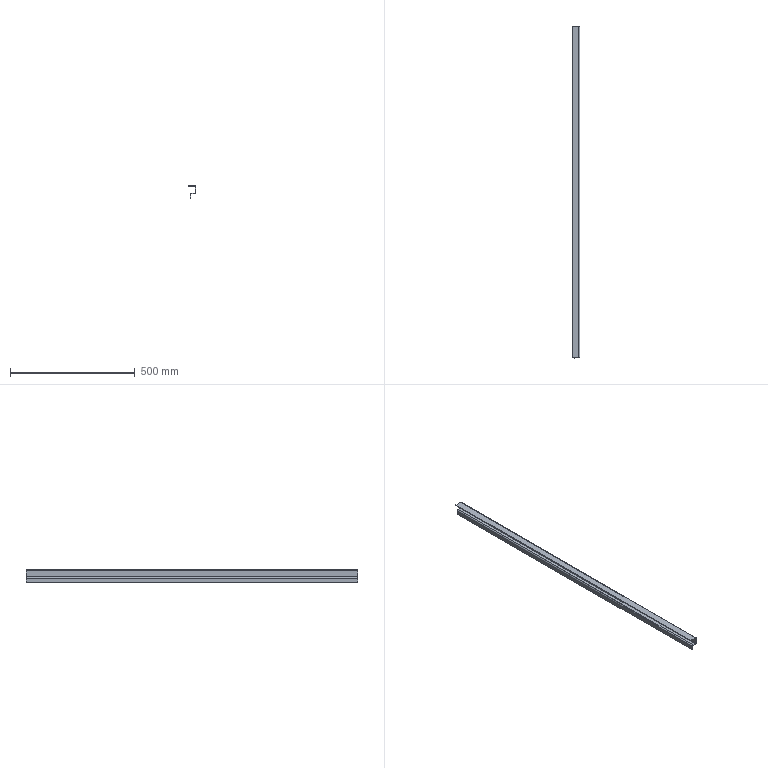Component | SolidWorks | BoxWelding-1_SupportPlate2.2-1 | 1 solid | 18 faces | box 31 x 1331 x 51 mm | volume 252490 mm3 | plane 12 | cylinder 6 | commonest cylinder face diameters 6 x3 10 x3
build123d program:
from build123d import *

# Parameters (mm, degrees)
EXTRUDE_THIN1_DEPTH = 665.5


with BuildPart() as part:
    # Sketch1 → Extrude-Thin1 (new, symmetric)
    with BuildSketch(Plane.XY):
        with BuildLine():
            Line((-1, 30), (-1, 4))
            ThreePointArc((-1, 4), (-1.879, 1.879), (-4, 1))
            Line((-4, 1), (-26, 1))
            ThreePointArc((-26, 1), (-28.121, 1.879), (-29, 4))
            Line((-29, 4), (-29, 16))
            ThreePointArc((-29, 16), (-30.464, 19.536), (-34, 21))
            Line((-34, 21), (-50, 21))
            Line((-50, 21), (-50, 19))
            Line((-50, 19), (-34, 19))
            ThreePointArc((-34, 19), (-31.879, 18.121), (-31, 16))
            Line((-31, 16), (-31, 4))
            ThreePointArc((-31, 4), (-29.536, 0.4645), (-26, -1))
            Line((-26, -1), (-4, -1))
            ThreePointArc((-4, -1), (-0.4645, 0.4645), (1, 4))
            Line((1, 4), (1, 30))
            Line((1, 30), (-1, 30))
        make_face()
    extrude(amount=EXTRUDE_THIN1_DEPTH, both=True)


solid = part.part

# Placed as in the assembly
solid = solid.moved(Location((450.622, 621.001, 379.013), (90, 0, 90)))
STEP:
#1=CARTESIAN_POINT('',(17.584,50.65,14.961));
#2=VERTEX_POINT('',#1);
#3=CARTESIAN_POINT('',(16.56,50.65,14.961));
#4=VERTEX_POINT('',#3);
#5=CARTESIAN_POINT('',(17.584,50.65,14.961));
#6=DIRECTION('',(-1.,-0.,-0.));
#7=VECTOR('',#6,39.37);
#8=LINE('',#5,#7);
#9=EDGE_CURVE('',#2,#4,#8,.T.);
#10=ORIENTED_EDGE('',*,*,#9,.T.);
#11=CARTESIAN_POINT('',(16.56,-1.752,14.961));
#12=VERTEX_POINT('',#11);
#13=CARTESIAN_POINT('',(16.56,-1.752,14.961));
#14=DIRECTION('',(-0.,1.,-0.));
#15=VECTOR('',#14,39.37);
#16=LINE('',#13,#15);
#17=EDGE_CURVE('',#12,#4,#16,.T.);
#18=ORIENTED_EDGE('',*,*,#17,.F.);
#19=CARTESIAN_POINT('',(17.584,-1.752,14.961));
#20=VERTEX_POINT('',#19);
#21=CARTESIAN_POINT('',(17.584,-1.752,14.961));
#22=DIRECTION('',(-1.,-0.,-0.));
#23=VECTOR('',#22,39.37);
#24=LINE('',#21,#23);
#25=EDGE_CURVE('',#20,#12,#24,.T.);
#26=ORIENTED_EDGE('',*,*,#25,.F.);
#27=CARTESIAN_POINT('',(17.584,-1.752,14.961));
#28=DIRECTION('',(-0.,1.,-0.));
#29=VECTOR('',#28,39.37);
#30=LINE('',#27,#29);
#31=EDGE_CURVE('',#20,#2,#30,.T.);
#32=ORIENTED_EDGE('',*,*,#31,.T.);
#33=EDGE_LOOP('',(#10,#18,#26,#32));
#34=FACE_OUTER_BOUND('',#33,.T.);
#35=CARTESIAN_POINT('',(17.584,-1.752,14.961));
#36=DIRECTION('',(0.,-0.,-1.));
#37=DIRECTION('',(0.,-1.,0.));
#38=AXIS2_PLACEMENT_3D('',#35,#36,#37);
#39=PLANE('',#38);
#40=ADVANCED_FACE('',(#34),#39,.F.);
#41=CARTESIAN_POINT('',(16.56,50.65,14.882));
#42=VERTEX_POINT('',#41);
#43=CARTESIAN_POINT('',(16.56,50.65,14.882));
#44=DIRECTION('',(-0.,0.,1.));
#45=VECTOR('',#44,39.37);
#46=LINE('',#43,#45);
#47=EDGE_CURVE('',#42,#4,#46,.T.);
#48=ORIENTED_EDGE('',*,*,#47,.F.);
#49=CARTESIAN_POINT('',(16.56,-1.752,14.882));
#50=VERTEX_POINT('',#49);
#51=CARTESIAN_POINT('',(16.56,-1.752,14.882));
#52=DIRECTION('',(-0.,1.,-0.));
#53=VECTOR('',#52,39.37);
#54=LINE('',#51,#53);
#55=EDGE_CURVE('',#50,#42,#54,.T.);
#56=ORIENTED_EDGE('',*,*,#55,.F.);
#57=CARTESIAN_POINT('',(16.56,-1.752,14.882));
#58=DIRECTION('',(-0.,0.,1.));
#59=VECTOR('',#58,39.37);
#60=LINE('',#57,#59);
#61=EDGE_CURVE('',#50,#12,#60,.T.);
#62=ORIENTED_EDGE('',*,*,#61,.T.);
#63=ORIENTED_EDGE('',*,*,#17,.T.);
#64=EDGE_LOOP('',(#48,#56,#62,#63));
#65=FACE_OUTER_BOUND('',#64,.T.);
#66=CARTESIAN_POINT('',(16.56,-1.752,14.882));
#67=DIRECTION('',(-1.,-0.,-0.));
#68=DIRECTION('',(0.,-1.,0.));
#69=AXIS2_PLACEMENT_3D('',#66,#67,#68);
#70=PLANE('',#69);
#71=ADVANCED_FACE('',(#65),#70,.T.);
#72=CARTESIAN_POINT('',(17.584,50.65,14.882));
#73=VERTEX_POINT('',#72);
#74=CARTESIAN_POINT('',(17.584,50.65,14.882));
#75=DIRECTION('',(-1.,-0.,-0.));
#76=VECTOR('',#75,39.37);
#77=LINE('',#74,#76);
#78=EDGE_CURVE('',#73,#42,#77,.T.);
#79=ORIENTED_EDGE('',*,*,#78,.F.);
#80=CARTESIAN_POINT('',(17.584,-1.752,14.882));
#81=VERTEX_POINT('',#80);
#82=CARTESIAN_POINT('',(17.584,-1.752,14.882));
#83=DIRECTION('',(-0.,1.,-0.));
#84=VECTOR('',#83,39.37);
#85=LINE('',#82,#84);
#86=EDGE_CURVE('',#81,#73,#85,.T.);
#87=ORIENTED_EDGE('',*,*,#86,.F.);
#88=CARTESIAN_POINT('',(17.584,-1.752,14.882));
#89=DIRECTION('',(-1.,-0.,-0.));
#90=VECTOR('',#89,39.37);
#91=LINE('',#88,#90);
#92=EDGE_CURVE('',#81,#50,#91,.T.);
#93=ORIENTED_EDGE('',*,*,#92,.T.);
#94=ORIENTED_EDGE('',*,*,#55,.T.);
#95=EDGE_LOOP('',(#79,#87,#93,#94));
#96=FACE_OUTER_BOUND('',#95,.T.);
#97=CARTESIAN_POINT('',(17.584,-1.752,14.882));
#98=DIRECTION('',(0.,-0.,-1.));
#99=DIRECTION('',(0.,-1.,0.));
#100=AXIS2_PLACEMENT_3D('',#97,#98,#99);
#101=PLANE('',#100);
#102=ADVANCED_FACE('',(#96),#101,.T.);
#103=CARTESIAN_POINT('',(17.702,50.65,14.764));
#104=VERTEX_POINT('',#103);
#105=CARTESIAN_POINT('',(17.584,50.65,14.764));
#106=DIRECTION('',(0.,-1.,0.));
#107=DIRECTION('',(0.,0.,1.));
#108=AXIS2_PLACEMENT_3D('',#105,#106,#107);
#109=CIRCLE('',#108,0.1181);
#110=EDGE_CURVE('',#104,#73,#109,.T.);
#111=ORIENTED_EDGE('',*,*,#110,.F.);
#112=CARTESIAN_POINT('',(17.702,-1.752,14.764));
#113=VERTEX_POINT('',#112);
#114=CARTESIAN_POINT('',(17.702,-1.752,14.764));
#115=DIRECTION('',(-0.,1.,-0.));
#116=VECTOR('',#115,39.37);
#117=LINE('',#114,#116);
#118=EDGE_CURVE('',#113,#104,#117,.T.);
#119=ORIENTED_EDGE('',*,*,#118,.F.);
#120=CARTESIAN_POINT('',(17.584,-1.752,14.764));
#121=DIRECTION('',(0.,-1.,0.));
#122=DIRECTION('',(0.,0.,1.));
#123=AXIS2_PLACEMENT_3D('',#120,#121,#122);
#124=CIRCLE('',#123,0.1181);
#125=EDGE_CURVE('',#113,#81,#124,.T.);
#126=ORIENTED_EDGE('',*,*,#125,.T.);
#127=ORIENTED_EDGE('',*,*,#86,.T.);
#128=EDGE_LOOP('',(#111,#119,#126,#127));
#129=FACE_OUTER_BOUND('',#128,.T.);
#130=CARTESIAN_POINT('',(17.584,-1.752,14.764));
#131=DIRECTION('',(-0.,1.,-0.));
#132=DIRECTION('',(0.,-0.,-1.));
#133=AXIS2_PLACEMENT_3D('',#130,#131,#132);
#134=CYLINDRICAL_SURFACE('',#133,0.1181);
#135=ADVANCED_FACE('',(#129),#134,.F.);
#136=CARTESIAN_POINT('',(17.702,50.65,13.898));
#137=VERTEX_POINT('',#136);
#138=CARTESIAN_POINT('',(17.702,50.65,14.764));
#139=DIRECTION('',(-0.,0.,1.));
#140=VECTOR('',#139,39.37);
#141=LINE('',#138,#140);
#142=EDGE_CURVE('',#137,#104,#141,.T.);
#143=ORIENTED_EDGE('',*,*,#142,.F.);
#144=CARTESIAN_POINT('',(17.702,-1.752,13.898));
#145=VERTEX_POINT('',#144);
#146=CARTESIAN_POINT('',(17.702,-1.752,13.898));
#147=DIRECTION('',(-0.,1.,-0.));
#148=VECTOR('',#147,39.37);
#149=LINE('',#146,#148);
#150=EDGE_CURVE('',#145,#137,#149,.T.);
#151=ORIENTED_EDGE('',*,*,#150,.F.);
#152=CARTESIAN_POINT('',(17.702,-1.752,14.764));
#153=DIRECTION('',(-0.,0.,1.));
#154=VECTOR('',#153,39.37);
#155=LINE('',#152,#154);
#156=EDGE_CURVE('',#145,#113,#155,.T.);
#157=ORIENTED_EDGE('',*,*,#156,.T.);
#158=ORIENTED_EDGE('',*,*,#118,.T.);
#159=EDGE_LOOP('',(#143,#151,#157,#158));
#160=FACE_OUTER_BOUND('',#159,.T.);
#161=CARTESIAN_POINT('',(17.702,-1.752,14.764));
#162=DIRECTION('',(-1.,-0.,-0.));
#163=DIRECTION('',(0.,-1.,0.));
#164=AXIS2_PLACEMENT_3D('',#161,#162,#163);
#165=PLANE('',#164);
#166=ADVANCED_FACE('',(#160),#165,.T.);
#167=CARTESIAN_POINT('',(17.584,50.65,13.78));
#168=VERTEX_POINT('',#167);
#169=CARTESIAN_POINT('',(17.584,50.65,13.898));
#170=DIRECTION('',(0.,-1.,0.));
#171=DIRECTION('',(0.,0.,1.));
#172=AXIS2_PLACEMENT_3D('',#169,#170,#171);
#173=CIRCLE('',#172,0.1181);
#174=EDGE_CURVE('',#168,#137,#173,.T.);
#175=ORIENTED_EDGE('',*,*,#174,.F.);
#176=CARTESIAN_POINT('',(17.584,-1.752,13.78));
#177=VERTEX_POINT('',#176);
#178=CARTESIAN_POINT('',(17.584,-1.752,13.78));
#179=DIRECTION('',(-0.,1.,-0.));
#180=VECTOR('',#179,39.37);
#181=LINE('',#178,#180);
#182=EDGE_CURVE('',#177,#168,#181,.T.);
#183=ORIENTED_EDGE('',*,*,#182,.F.);
#184=CARTESIAN_POINT('',(17.584,-1.752,13.898));
#185=DIRECTION('',(0.,-1.,0.));
#186=DIRECTION('',(0.,0.,1.));
#187=AXIS2_PLACEMENT_3D('',#184,#185,#186);
#188=CIRCLE('',#187,0.1181);
#189=EDGE_CURVE('',#177,#145,#188,.T.);
#190=ORIENTED_EDGE('',*,*,#189,.T.);
#191=ORIENTED_EDGE('',*,*,#150,.T.);
#192=EDGE_LOOP('',(#175,#183,#190,#191));
#193=FACE_OUTER_BOUND('',#192,.T.);
#194=CARTESIAN_POINT('',(17.584,-1.752,13.898));
#195=DIRECTION('',(-0.,1.,-0.));
#196=DIRECTION('',(0.,-0.,-1.));
#197=AXIS2_PLACEMENT_3D('',#194,#195,#196);
#198=CYLINDRICAL_SURFACE('',#197,0.1181);
#199=ADVANCED_FACE('',(#193),#198,.F.);
#200=CARTESIAN_POINT('',(17.111,50.65,13.78));
#201=VERTEX_POINT('',#200);
#202=CARTESIAN_POINT('',(17.584,50.65,13.78));
#203=DIRECTION('',(1.,0.,0.));
#204=VECTOR('',#203,39.37);
#205=LINE('',#202,#204);
#206=EDGE_CURVE('',#201,#168,#205,.T.);
#207=ORIENTED_EDGE('',*,*,#206,.F.);
#208=CARTESIAN_POINT('',(17.111,-1.752,13.78));
#209=VERTEX_POINT('',#208);
#210=CARTESIAN_POINT('',(17.111,-1.752,13.78));
#211=DIRECTION('',(-0.,1.,-0.));
#212=VECTOR('',#211,39.37);
#213=LINE('',#210,#212);
#214=EDGE_CURVE('',#209,#201,#213,.T.);
#215=ORIENTED_EDGE('',*,*,#214,.F.);
#216=CARTESIAN_POINT('',(17.584,-1.752,13.78));
#217=DIRECTION('',(1.,0.,0.));
#218=VECTOR('',#217,39.37);
#219=LINE('',#216,#218);
#220=EDGE_CURVE('',#209,#177,#219,.T.);
#221=ORIENTED_EDGE('',*,*,#220,.T.);
#222=ORIENTED_EDGE('',*,*,#182,.T.);
#223=EDGE_LOOP('',(#207,#215,#221,#222));
#224=FACE_OUTER_BOUND('',#223,.T.);
#225=CARTESIAN_POINT('',(17.584,-1.752,13.78));
#226=DIRECTION('',(-0.,0.,1.));
#227=DIRECTION('',(-0.,1.,-0.));
#228=AXIS2_PLACEMENT_3D('',#225,#226,#227);
#229=PLANE('',#228);
#230=ADVANCED_FACE('',(#224),#229,.T.);
#231=CARTESIAN_POINT('',(16.914,50.65,13.583));
#232=VERTEX_POINT('',#231);
#233=CARTESIAN_POINT('',(17.111,50.65,13.583));
#234=DIRECTION('',(-0.,1.,-0.));
#235=DIRECTION('',(0.,0.,1.));
#236=AXIS2_PLACEMENT_3D('',#233,#234,#235);
#237=CIRCLE('',#236,0.1969);
#238=EDGE_CURVE('',#232,#201,#237,.T.);
#239=ORIENTED_EDGE('',*,*,#238,.F.);
#240=CARTESIAN_POINT('',(16.914,-1.752,13.583));
#241=VERTEX_POINT('',#240);
#242=CARTESIAN_POINT('',(16.914,-1.752,13.583));
#243=DIRECTION('',(-0.,1.,-0.));
#244=VECTOR('',#243,39.37);
#245=LINE('',#242,#244);
#246=EDGE_CURVE('',#241,#232,#245,.T.);
#247=ORIENTED_EDGE('',*,*,#246,.F.);
#248=CARTESIAN_POINT('',(17.111,-1.752,13.583));
#249=DIRECTION('',(-0.,1.,-0.));
#250=DIRECTION('',(-0.,0.,1.));
#251=AXIS2_PLACEMENT_3D('',#248,#249,#250);
#252=CIRCLE('',#251,0.1969);
#253=EDGE_CURVE('',#241,#209,#252,.T.);
#254=ORIENTED_EDGE('',*,*,#253,.T.);
#255=ORIENTED_EDGE('',*,*,#214,.T.);
#256=EDGE_LOOP('',(#239,#247,#254,#255));
#257=FACE_OUTER_BOUND('',#256,.T.);
#258=CARTESIAN_POINT('',(17.111,-1.752,13.583));
#259=DIRECTION('',(-0.,1.,-0.));
#260=DIRECTION('',(0.,-0.,-1.));
#261=AXIS2_PLACEMENT_3D('',#258,#259,#260);
#262=CYLINDRICAL_SURFACE('',#261,0.1969);
#263=ADVANCED_FACE('',(#257),#262,.T.);
#264=CARTESIAN_POINT('',(16.914,50.65,12.953));
#265=VERTEX_POINT('',#264);
#266=CARTESIAN_POINT('',(16.914,50.65,13.583));
#267=DIRECTION('',(-0.,0.,1.));
#268=VECTOR('',#267,39.37);
#269=LINE('',#266,#268);
#270=EDGE_CURVE('',#265,#232,#269,.T.);
#271=ORIENTED_EDGE('',*,*,#270,.F.);
#272=CARTESIAN_POINT('',(16.914,-1.752,12.953));
#273=VERTEX_POINT('',#272);
#274=CARTESIAN_POINT('',(16.914,-1.752,12.953));
#275=DIRECTION('',(-0.,1.,-0.));
#276=VECTOR('',#275,39.37);
#277=LINE('',#274,#276);
#278=EDGE_CURVE('',#273,#265,#277,.T.);
#279=ORIENTED_EDGE('',*,*,#278,.F.);
#280=CARTESIAN_POINT('',(16.914,-1.752,13.583));
#281=DIRECTION('',(-0.,0.,1.));
#282=VECTOR('',#281,39.37);
#283=LINE('',#280,#282);
#284=EDGE_CURVE('',#273,#241,#283,.T.);
#285=ORIENTED_EDGE('',*,*,#284,.T.);
#286=ORIENTED_EDGE('',*,*,#246,.T.);
#287=EDGE_LOOP('',(#271,#279,#285,#286));
#288=FACE_OUTER_BOUND('',#287,.T.);
#289=CARTESIAN_POINT('',(16.914,-1.752,13.583));
#290=DIRECTION('',(-1.,-0.,-0.));
#291=DIRECTION('',(0.,-0.,-1.));
#292=AXIS2_PLACEMENT_3D('',#289,#290,#291);
#293=PLANE('',#292);
#294=ADVANCED_FACE('',(#288),#293,.T.);
#295=CARTESIAN_POINT('',(16.993,50.65,12.953));
#296=VERTEX_POINT('',#295);
#297=CARTESIAN_POINT('',(16.993,50.65,12.953));
#298=DIRECTION('',(-1.,-0.,-0.));
#299=VECTOR('',#298,39.37);
#300=LINE('',#297,#299);
#301=EDGE_CURVE('',#296,#265,#300,.T.);
#302=ORIENTED_EDGE('',*,*,#301,.F.);
#303=CARTESIAN_POINT('',(16.993,-1.752,12.953));
#304=VERTEX_POINT('',#303);
#305=CARTESIAN_POINT('',(16.993,-1.752,12.953));
#306=DIRECTION('',(-0.,1.,-0.));
#307=VECTOR('',#306,39.37);
#308=LINE('',#305,#307);
#309=EDGE_CURVE('',#304,#296,#308,.T.);
#310=ORIENTED_EDGE('',*,*,#309,.F.);
#311=CARTESIAN_POINT('',(16.993,-1.752,12.953));
#312=DIRECTION('',(-1.,-0.,-0.));
#313=VECTOR('',#312,39.37);
#314=LINE('',#311,#313);
#315=EDGE_CURVE('',#304,#273,#314,.T.);
#316=ORIENTED_EDGE('',*,*,#315,.T.);
#317=ORIENTED_EDGE('',*,*,#278,.T.);
#318=EDGE_LOOP('',(#302,#310,#316,#317));
#319=FACE_OUTER_BOUND('',#318,.T.);
#320=CARTESIAN_POINT('',(16.993,-1.752,12.953));
#321=DIRECTION('',(0.,-0.,-1.));
#322=DIRECTION('',(0.,-1.,0.));
#323=AXIS2_PLACEMENT_3D('',#320,#321,#322);
#324=PLANE('',#323);
#325=ADVANCED_FACE('',(#319),#324,.T.);
#326=CARTESIAN_POINT('',(16.993,50.65,13.583));
#327=VERTEX_POINT('',#326);
#328=CARTESIAN_POINT('',(16.993,50.65,13.583));
#329=DIRECTION('',(-0.,0.,1.));
#330=VECTOR('',#329,39.37);
#331=LINE('',#328,#330);
#332=EDGE_CURVE('',#296,#327,#331,.T.);
#333=ORIENTED_EDGE('',*,*,#332,.T.);
#334=CARTESIAN_POINT('',(16.993,-1.752,13.583));
#335=VERTEX_POINT('',#334);
#336=CARTESIAN_POINT('',(16.993,-1.752,13.583));
#337=DIRECTION('',(-0.,1.,-0.));
#338=VECTOR('',#337,39.37);
#339=LINE('',#336,#338);
#340=EDGE_CURVE('',#335,#327,#339,.T.);
#341=ORIENTED_EDGE('',*,*,#340,.F.);
#342=CARTESIAN_POINT('',(16.993,-1.752,13.583));
#343=DIRECTION('',(-0.,0.,1.));
#344=VECTOR('',#343,39.37);
#345=LINE('',#342,#344);
#346=EDGE_CURVE('',#304,#335,#345,.T.);
#347=ORIENTED_EDGE('',*,*,#346,.F.);
#348=ORIENTED_EDGE('',*,*,#309,.T.);
#349=EDGE_LOOP('',(#333,#341,#347,#348));
#350=FACE_OUTER_BOUND('',#349,.T.);
#351=CARTESIAN_POINT('',(16.993,-1.752,13.583));
#352=DIRECTION('',(-1.,-0.,-0.));
#353=DIRECTION('',(0.,-0.,-1.));
#354=AXIS2_PLACEMENT_3D('',#351,#352,#353);
#355=PLANE('',#354);
#356=ADVANCED_FACE('',(#350),#355,.F.);
#357=CARTESIAN_POINT('',(17.111,50.65,13.701));
#358=VERTEX_POINT('',#357);
#359=CARTESIAN_POINT('',(17.111,50.65,13.583));
#360=DIRECTION('',(-0.,1.,-0.));
#361=DIRECTION('',(0.,0.,1.));
#362=AXIS2_PLACEMENT_3D('',#359,#360,#361);
#363=CIRCLE('',#362,0.1181);
#364=EDGE_CURVE('',#327,#358,#363,.T.);
#365=ORIENTED_EDGE('',*,*,#364,.T.);
#366=CARTESIAN_POINT('',(17.111,-1.752,13.701));
#367=VERTEX_POINT('',#366);
#368=CARTESIAN_POINT('',(17.111,-1.752,13.701));
#369=DIRECTION('',(-0.,1.,-0.));
#370=VECTOR('',#369,39.37);
#371=LINE('',#368,#370);
#372=EDGE_CURVE('',#367,#358,#371,.T.);
#373=ORIENTED_EDGE('',*,*,#372,.F.);
#374=CARTESIAN_POINT('',(17.111,-1.752,13.583));
#375=DIRECTION('',(-0.,1.,-0.));
#376=DIRECTION('',(-0.,0.,1.));
#377=AXIS2_PLACEMENT_3D('',#374,#375,#376);
#378=CIRCLE('',#377,0.1181);
#379=EDGE_CURVE('',#335,#367,#378,.T.);
#380=ORIENTED_EDGE('',*,*,#379,.F.);
#381=ORIENTED_EDGE('',*,*,#340,.T.);
#382=EDGE_LOOP('',(#365,#373,#380,#381));
#383=FACE_OUTER_BOUND('',#382,.T.);
#384=CARTESIAN_POINT('',(17.111,-1.752,13.583));
#385=DIRECTION('',(-0.,1.,-0.));
#386=DIRECTION('',(0.,-0.,-1.));
#387=AXIS2_PLACEMENT_3D('',#384,#385,#386);
#388=CYLINDRICAL_SURFACE('',#387,0.1181);
#389=ADVANCED_FACE('',(#383),#388,.F.);
#390=CARTESIAN_POINT('',(17.584,50.65,13.701));
#391=VERTEX_POINT('',#390);
#392=CARTESIAN_POINT('',(17.584,50.65,13.701));
#393=DIRECTION('',(1.,0.,0.));
#394=VECTOR('',#393,39.37);
#395=LINE('',#392,#394);
#396=EDGE_CURVE('',#358,#391,#395,.T.);
#397=ORIENTED_EDGE('',*,*,#396,.T.);
#398=CARTESIAN_POINT('',(17.584,-1.752,13.701));
#399=VERTEX_POINT('',#398);
#400=CARTESIAN_POINT('',(17.584,-1.752,13.701));
#401=DIRECTION('',(-0.,1.,-0.));
#402=VECTOR('',#401,39.37);
#403=LINE('',#400,#402);
#404=EDGE_CURVE('',#399,#391,#403,.T.);
#405=ORIENTED_EDGE('',*,*,#404,.F.);
#406=CARTESIAN_POINT('',(17.584,-1.752,13.701));
#407=DIRECTION('',(1.,0.,0.));
#408=VECTOR('',#407,39.37);
#409=LINE('',#406,#408);
#410=EDGE_CURVE('',#367,#399,#409,.T.);
#411=ORIENTED_EDGE('',*,*,#410,.F.);
#412=ORIENTED_EDGE('',*,*,#372,.T.);
#413=EDGE_LOOP('',(#397,#405,#411,#412));
#414=FACE_OUTER_BOUND('',#413,.T.);
#415=CARTESIAN_POINT('',(17.584,-1.752,13.701));
#416=DIRECTION('',(-0.,0.,1.));
#417=DIRECTION('',(-0.,1.,-0.));
#418=AXIS2_PLACEMENT_3D('',#415,#416,#417);
#419=PLANE('',#418);
#420=ADVANCED_FACE('',(#414),#419,.F.);
#421=CARTESIAN_POINT('',(17.78,50.65,13.898));
#422=VERTEX_POINT('',#421);
#423=CARTESIAN_POINT('',(17.584,50.65,13.898));
#424=DIRECTION('',(0.,-1.,0.));
#425=DIRECTION('',(0.,0.,1.));
#426=AXIS2_PLACEMENT_3D('',#423,#424,#425);
#427=CIRCLE('',#426,0.1969);
#428=EDGE_CURVE('',#391,#422,#427,.T.);
#429=ORIENTED_EDGE('',*,*,#428,.T.);
#430=CARTESIAN_POINT('',(17.78,-1.752,13.898));
#431=VERTEX_POINT('',#430);
#432=CARTESIAN_POINT('',(17.78,-1.752,13.898));
#433=DIRECTION('',(-0.,1.,-0.));
#434=VECTOR('',#433,39.37);
#435=LINE('',#432,#434);
#436=EDGE_CURVE('',#431,#422,#435,.T.);
#437=ORIENTED_EDGE('',*,*,#436,.F.);
#438=CARTESIAN_POINT('',(17.584,-1.752,13.898));
#439=DIRECTION('',(0.,-1.,0.));
#440=DIRECTION('',(0.,0.,1.));
#441=AXIS2_PLACEMENT_3D('',#438,#439,#440);
#442=CIRCLE('',#441,0.1969);
#443=EDGE_CURVE('',#399,#431,#442,.T.);
#444=ORIENTED_EDGE('',*,*,#443,.F.);
#445=ORIENTED_EDGE('',*,*,#404,.T.);
#446=EDGE_LOOP('',(#429,#437,#444,#445));
#447=FACE_OUTER_BOUND('',#446,.T.);
#448=CARTESIAN_POINT('',(17.584,-1.752,13.898));
#449=DIRECTION('',(-0.,1.,-0.));
#450=DIRECTION('',(0.,-0.,-1.));
#451=AXIS2_PLACEMENT_3D('',#448,#449,#450);
#452=CYLINDRICAL_SURFACE('',#451,0.1969);
#453=ADVANCED_FACE('',(#447),#452,.T.);
#454=CARTESIAN_POINT('',(17.78,50.65,14.764));
#455=VERTEX_POINT('',#454);
#456=CARTESIAN_POINT('',(17.78,50.65,14.764));
#457=DIRECTION('',(-0.,0.,1.));
#458=VECTOR('',#457,39.37);
#459=LINE('',#456,#458);
#460=EDGE_CURVE('',#422,#455,#459,.T.);
#461=ORIENTED_EDGE('',*,*,#460,.T.);
#462=CARTESIAN_POINT('',(17.78,-1.752,14.764));
#463=VERTEX_POINT('',#462);
#464=CARTESIAN_POINT('',(17.78,-1.752,14.764));
#465=DIRECTION('',(-0.,1.,-0.));
#466=VECTOR('',#465,39.37);
#467=LINE('',#464,#466);
#468=EDGE_CURVE('',#463,#455,#467,.T.);
#469=ORIENTED_EDGE('',*,*,#468,.F.);
#470=CARTESIAN_POINT('',(17.78,-1.752,14.764));
#471=DIRECTION('',(-0.,0.,1.));
#472=VECTOR('',#471,39.37);
#473=LINE('',#470,#472);
#474=EDGE_CURVE('',#431,#463,#473,.T.);
#475=ORIENTED_EDGE('',*,*,#474,.F.);
#476=ORIENTED_EDGE('',*,*,#436,.T.);
#477=EDGE_LOOP('',(#461,#469,#475,#476));
#478=FACE_OUTER_BOUND('',#477,.T.);
#479=CARTESIAN_POINT('',(17.78,-1.752,14.764));
#480=DIRECTION('',(-1.,-0.,-0.));
#481=DIRECTION('',(0.,-1.,0.));
#482=AXIS2_PLACEMENT_3D('',#479,#480,#481);
#483=PLANE('',#482);
#484=ADVANCED_FACE('',(#478),#483,.F.);
#485=CARTESIAN_POINT('',(17.584,50.65,14.764));
#486=DIRECTION('',(0.,-1.,0.));
#487=DIRECTION('',(0.,0.,1.));
#488=AXIS2_PLACEMENT_3D('',#485,#486,#487);
#489=CIRCLE('',#488,0.1969);
#490=EDGE_CURVE('',#455,#2,#489,.T.);
#491=ORIENTED_EDGE('',*,*,#490,.T.);
#492=ORIENTED_EDGE('',*,*,#31,.F.);
#493=CARTESIAN_POINT('',(17.584,-1.752,14.764));
#494=DIRECTION('',(0.,-1.,0.));
#495=DIRECTION('',(0.,0.,1.));
#496=AXIS2_PLACEMENT_3D('',#493,#494,#495);
#497=CIRCLE('',#496,0.1969);
#498=EDGE_CURVE('',#463,#20,#497,.T.);
#499=ORIENTED_EDGE('',*,*,#498,.F.);
#500=ORIENTED_EDGE('',*,*,#468,.T.);
#501=EDGE_LOOP('',(#491,#492,#499,#500));
#502=FACE_OUTER_BOUND('',#501,.T.);
#503=CARTESIAN_POINT('',(17.584,-1.752,14.764));
#504=DIRECTION('',(-0.,1.,-0.));
#505=DIRECTION('',(0.,-0.,-1.));
#506=AXIS2_PLACEMENT_3D('',#503,#504,#505);
#507=CYLINDRICAL_SURFACE('',#506,0.1969);
#508=ADVANCED_FACE('',(#502),#507,.T.);
#509=ORIENTED_EDGE('',*,*,#25,.T.);
#510=ORIENTED_EDGE('',*,*,#61,.F.);
#511=ORIENTED_EDGE('',*,*,#92,.F.);
#512=ORIENTED_EDGE('',*,*,#125,.F.);
#513=ORIENTED_EDGE('',*,*,#156,.F.);
#514=ORIENTED_EDGE('',*,*,#189,.F.);
#515=ORIENTED_EDGE('',*,*,#220,.F.);
#516=ORIENTED_EDGE('',*,*,#253,.F.);
#517=ORIENTED_EDGE('',*,*,#284,.F.);
#518=ORIENTED_EDGE('',*,*,#315,.F.);
#519=ORIENTED_EDGE('',*,*,#346,.T.);
#520=ORIENTED_EDGE('',*,*,#379,.T.);
#521=ORIENTED_EDGE('',*,*,#410,.T.);
#522=ORIENTED_EDGE('',*,*,#443,.T.);
#523=ORIENTED_EDGE('',*,*,#474,.T.);
#524=ORIENTED_EDGE('',*,*,#498,.T.);
#525=EDGE_LOOP('',(#509,#510,#511,#512,#513,#514,#515,#516,#517,#518,#519,#520,#521,#522,#523,#524));
#526=FACE_OUTER_BOUND('',#525,.T.);
#527=CARTESIAN_POINT('',(17.584,-1.752,14.764));
#528=DIRECTION('',(0.,-1.,0.));
#529=DIRECTION('',(-0.,0.,1.));
#530=AXIS2_PLACEMENT_3D('',#527,#528,#529);
#531=PLANE('',#530);
#532=ADVANCED_FACE('',(#526),#531,.T.);
#533=ORIENTED_EDGE('',*,*,#9,.F.);
#534=ORIENTED_EDGE('',*,*,#490,.F.);
#535=ORIENTED_EDGE('',*,*,#460,.F.);
#536=ORIENTED_EDGE('',*,*,#428,.F.);
#537=ORIENTED_EDGE('',*,*,#396,.F.);
#538=ORIENTED_EDGE('',*,*,#364,.F.);
#539=ORIENTED_EDGE('',*,*,#332,.F.);
#540=ORIENTED_EDGE('',*,*,#301,.T.);
#541=ORIENTED_EDGE('',*,*,#270,.T.);
#542=ORIENTED_EDGE('',*,*,#238,.T.);
#543=ORIENTED_EDGE('',*,*,#206,.T.);
#544=ORIENTED_EDGE('',*,*,#174,.T.);
#545=ORIENTED_EDGE('',*,*,#142,.T.);
#546=ORIENTED_EDGE('',*,*,#110,.T.);
#547=ORIENTED_EDGE('',*,*,#78,.T.);
#548=ORIENTED_EDGE('',*,*,#47,.T.);
#549=EDGE_LOOP('',(#533,#534,#535,#536,#537,#538,#539,#540,#541,#542,#543,#544,#545,#546,#547,#548));
#550=FACE_OUTER_BOUND('',#549,.T.);
#551=CARTESIAN_POINT('',(17.584,50.65,14.764));
#552=DIRECTION('',(0.,-1.,0.));
#553=DIRECTION('',(-0.,0.,1.));
#554=AXIS2_PLACEMENT_3D('',#551,#552,#553);
#555=PLANE('',#554);
#556=ADVANCED_FACE('',(#550),#555,.F.);
#557=CLOSED_SHELL('',(#40,#71,#102,#135,#166,#199,#230,#263,#294,#325,#356,#389,#420,#453,#484,#508,#532,#556));
#558=MANIFOLD_SOLID_BREP('',#557);
#559=CARTESIAN_POINT('',(0.,0.,0.));
#560=DIRECTION('',(0.,0.,1.));
#561=DIRECTION('',(1.,0.,0.));
#562=AXIS2_PLACEMENT_3D('',#559,#560,#561);
#563=(LENGTH_UNIT()NAMED_UNIT(*)SI_UNIT($,.METRE.));
#564=LENGTH_MEASURE_WITH_UNIT(LENGTH_MEASURE(0.0254),#563);
#565=DIMENSIONAL_EXPONENTS(1.,0.,0.,0.,0.,0.,0.);
#566=(CONVERSION_BASED_UNIT('',#564)LENGTH_UNIT()NAMED_UNIT(#565));
#567=UNCERTAINTY_MEASURE_WITH_UNIT(LENGTH_MEASURE(0.00001),#566,'','');
#568=(NAMED_UNIT(*)PLANE_ANGLE_UNIT()SI_UNIT($,.RADIAN.));
#569=(NAMED_UNIT(*)SI_UNIT($,.STERADIAN.)SOLID_ANGLE_UNIT());
#570=(GEOMETRIC_REPRESENTATION_CONTEXT(3)GLOBAL_UNCERTAINTY_ASSIGNED_CONTEXT((#567))GLOBAL_UNIT_ASSIGNED_CONTEXT((#566,#568,#569))REPRESENTATION_CONTEXT('',''));
#571=ADVANCED_BREP_SHAPE_REPRESENTATION('',(#558,#562),#570);
#572=COLOUR_RGB('',0.7922,0.8196,0.9333);
#573=FILL_AREA_STYLE_COLOUR('',#572);
#574=FILL_AREA_STYLE('',(#573));
#575=SURFACE_STYLE_FILL_AREA(#574);
#576=SURFACE_SIDE_STYLE('',(#575));
#577=SURFACE_STYLE_USAGE(.BOTH.,#576);
#578=PRESENTATION_STYLE_ASSIGNMENT((#577));
#579=STYLED_ITEM('',(#578),#558);
#580=PRESENTATION_LAYER_ASSIGNMENT('','',(#579));
#581=(LENGTH_UNIT()NAMED_UNIT(*)SI_UNIT($,.METRE.));
#582=LENGTH_MEASURE_WITH_UNIT(LENGTH_MEASURE(0.0254),#581);
#583=DIMENSIONAL_EXPONENTS(1.,0.,0.,0.,0.,0.,0.);
#584=(CONVERSION_BASED_UNIT('',#582)LENGTH_UNIT()NAMED_UNIT(#583));
#585=UNCERTAINTY_MEASURE_WITH_UNIT(LENGTH_MEASURE(0.00001),#584,'','');
#586=(NAMED_UNIT(*)PLANE_ANGLE_UNIT()SI_UNIT($,.RADIAN.));
#587=(NAMED_UNIT(*)SI_UNIT($,.STERADIAN.)SOLID_ANGLE_UNIT());
#588=(GEOMETRIC_REPRESENTATION_CONTEXT(3)GLOBAL_UNCERTAINTY_ASSIGNED_CONTEXT((#585))GLOBAL_UNIT_ASSIGNED_CONTEXT((#584,#586,#587))REPRESENTATION_CONTEXT('',''));
#589=MECHANICAL_DESIGN_GEOMETRIC_PRESENTATION_REPRESENTATION('',(#579),#588);